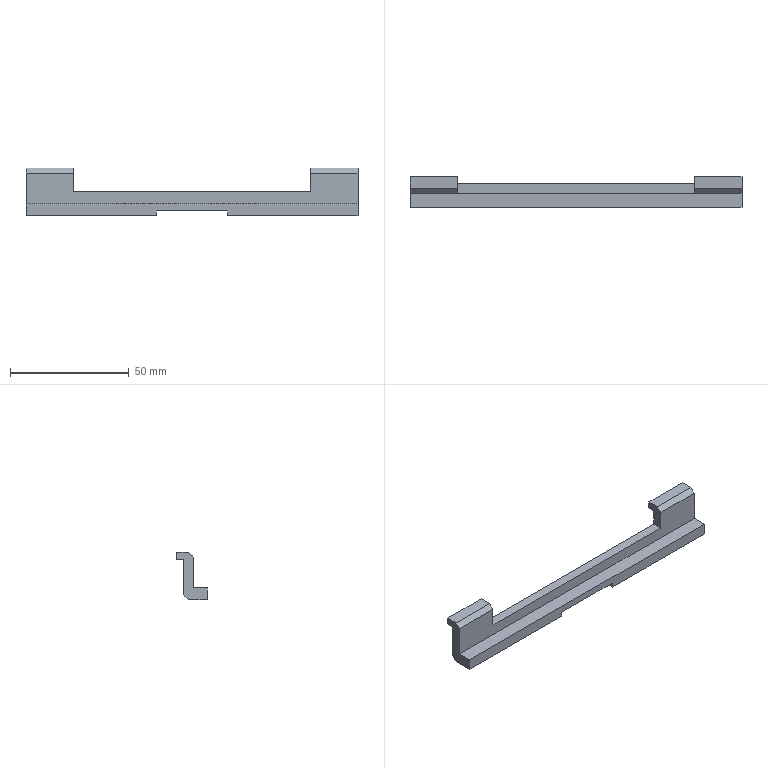Component | SolidWorks | Gripper-2024-3-4-07-1 | 1 solid | 24 faces | box 140 x 13 x 20 mm | volume 10860 mm3 | plane 24 | material S45C
build123d program:
from build123d import *

# Parameters (mm, degrees)
BOSS_EXTRUDE1_DEPTH = 140
SKETCH2_W           = 100
SKETCH2_H           = 10
CUT_EXTRUDE1_DEPTH  = 250
SKETCH3_W           = 10
SKETCH3_H           = 30
CUT_EXTRUDE2_DEPTH  = 2
SKETCH4_W           = 6
SKETCH4_H           = 15
CUT_EXTRUDE3_DEPTH  = 143.018
CHAMFER1_SIZE       = 2


with BuildPart() as part:
    # Sketch1 → Boss-Extrude1 (new body)
    with BuildSketch(Plane.XY):
        Polygon((0, 0), (-13, 0), (-13, 3), (-10, 3), (-10, 20), (0, 20), align=None)
    extrude(amount=BOSS_EXTRUDE1_DEPTH)

    # Sketch2 → Cut-Extrude1 (cut)
    with BuildSketch(Plane(origin=(0, 0, 0), x_dir=(0, 0, -1), z_dir=(1, 0, 0))):
        with Locations((-70, 5)):
            Rectangle(SKETCH2_W, SKETCH2_H)
    extrude(amount=-CUT_EXTRUDE1_DEPTH, mode=Mode.SUBTRACT)

    # Sketch3 → Cut-Extrude2 (cut)
    with BuildSketch(Plane(origin=(0, 20, 0), x_dir=(1, 0, 0), z_dir=(0, 1, 0))):
        with Locations((-5, -70)):
            Rectangle(SKETCH3_W, SKETCH3_H)
    extrude(amount=-CUT_EXTRUDE2_DEPTH, mode=Mode.SUBTRACT)

    # Sketch4 → Cut-Extrude3 (cut, through all)
    with BuildSketch(Plane.XY.offset(140)):
        with Locations((-3, 7.5)):
            Rectangle(SKETCH4_W, SKETCH4_H)
    extrude(amount=-CUT_EXTRUDE3_DEPTH, mode=Mode.SUBTRACT)

    # Chamfer1
    chamfer1_edges = [part.edges().sort_by_distance(p)[0] for p in [
        (-10, 20, 27.5),
        (-10, 20, 112.5),
        (-6, 0, 10),
        (-6, 0, 130),
    ]]
    chamfer(chamfer1_edges, length=CHAMFER1_SIZE)


solid = part.part

# Placed as in the assembly
solid = solid.moved(Location((-170.094, -141.769, 348), (-90, 90, 0)))
STEP:
#1=COLOUR_RGB('',0.7922,0.8196,0.9333);
#2=FILL_AREA_STYLE_COLOUR('',#1);
#3=FILL_AREA_STYLE('',(#2));
#4=SURFACE_STYLE_FILL_AREA(#3);
#5=SURFACE_SIDE_STYLE('',(#4));
#6=SURFACE_STYLE_USAGE(.BOTH.,#5);
#7=PRESENTATION_STYLE_ASSIGNMENT((#6));
#8=CARTESIAN_POINT('',(-6.697,-5.581,12.913));
#9=VERTEX_POINT('',#8);
#10=CARTESIAN_POINT('',(-6.697,-5.267,12.913));
#11=VERTEX_POINT('',#10);
#12=CARTESIAN_POINT('',(-6.697,-5.581,12.913));
#13=DIRECTION('',(-0.,1.,-0.));
#14=VECTOR('',#13,39.37);
#15=LINE('',#12,#14);
#16=EDGE_CURVE('',#9,#11,#15,.T.);
#17=ORIENTED_EDGE('',*,*,#16,.T.);
#18=CARTESIAN_POINT('',(-4.531,-5.267,12.913));
#19=VERTEX_POINT('',#18);
#20=CARTESIAN_POINT('',(-1.185,-5.267,12.913));
#21=DIRECTION('',(1.,-0.,0.));
#22=VECTOR('',#21,39.37);
#23=LINE('',#20,#22);
#24=EDGE_CURVE('',#11,#19,#23,.T.);
#25=ORIENTED_EDGE('',*,*,#24,.T.);
#26=CARTESIAN_POINT('',(-4.531,-5.581,12.913));
#27=VERTEX_POINT('',#26);
#28=CARTESIAN_POINT('',(-4.531,-5.581,12.913));
#29=DIRECTION('',(-0.,1.,-0.));
#30=VECTOR('',#29,39.37);
#31=LINE('',#28,#30);
#32=EDGE_CURVE('',#27,#19,#31,.T.);
#33=ORIENTED_EDGE('',*,*,#32,.F.);
#34=CARTESIAN_POINT('',(-1.185,-5.581,12.913));
#35=DIRECTION('',(-1.,0.,-0.));
#36=VECTOR('',#35,39.37);
#37=LINE('',#34,#36);
#38=EDGE_CURVE('',#27,#9,#37,.T.);
#39=ORIENTED_EDGE('',*,*,#38,.T.);
#40=EDGE_LOOP('',(#17,#25,#33,#39));
#41=FACE_OUTER_BOUND('',#40,.T.);
#42=CARTESIAN_POINT('',(-1.185,-5.581,12.913));
#43=DIRECTION('',(-0.,0.,1.));
#44=DIRECTION('',(0.,-1.,0.));
#45=AXIS2_PLACEMENT_3D('',#42,#43,#44);
#46=PLANE('',#45);
#47=ADVANCED_FACE('',(#41),#46,.F.);
#48=CARTESIAN_POINT('',(-1.185,-5.188,13.583));
#49=VERTEX_POINT('',#48);
#50=CARTESIAN_POINT('',(-1.972,-5.188,13.583));
#51=VERTEX_POINT('',#50);
#52=CARTESIAN_POINT('',(-1.185,-5.188,13.583));
#53=DIRECTION('',(-1.,0.,-0.));
#54=VECTOR('',#53,39.37);
#55=LINE('',#52,#54);
#56=EDGE_CURVE('',#49,#51,#55,.T.);
#57=ORIENTED_EDGE('',*,*,#56,.T.);
#58=CARTESIAN_POINT('',(-1.972,-5.07,13.583));
#59=VERTEX_POINT('',#58);
#60=CARTESIAN_POINT('',(-1.972,-5.07,13.583));
#61=DIRECTION('',(-0.,1.,-0.));
#62=VECTOR('',#61,39.37);
#63=LINE('',#60,#62);
#64=EDGE_CURVE('',#51,#59,#63,.T.);
#65=ORIENTED_EDGE('',*,*,#64,.T.);
#66=CARTESIAN_POINT('',(-1.185,-5.07,13.583));
#67=VERTEX_POINT('',#66);
#68=CARTESIAN_POINT('',(-1.185,-5.07,13.583));
#69=DIRECTION('',(-1.,0.,-0.));
#70=VECTOR('',#69,39.37);
#71=LINE('',#68,#70);
#72=EDGE_CURVE('',#67,#59,#71,.T.);
#73=ORIENTED_EDGE('',*,*,#72,.F.);
#74=CARTESIAN_POINT('',(-1.185,-5.07,13.583));
#75=DIRECTION('',(-0.,1.,-0.));
#76=VECTOR('',#75,39.37);
#77=LINE('',#74,#76);
#78=EDGE_CURVE('',#49,#67,#77,.T.);
#79=ORIENTED_EDGE('',*,*,#78,.F.);
#80=EDGE_LOOP('',(#57,#65,#73,#79));
#81=FACE_OUTER_BOUND('',#80,.T.);
#82=CARTESIAN_POINT('',(-1.185,-5.07,13.583));
#83=DIRECTION('',(-0.,0.,1.));
#84=DIRECTION('',(-1.,0.,-0.));
#85=AXIS2_PLACEMENT_3D('',#82,#83,#84);
#86=PLANE('',#85);
#87=ADVANCED_FACE('',(#81),#86,.F.);
#88=ORIENTED_EDGE('',*,*,#72,.T.);
#89=CARTESIAN_POINT('',(-1.972,-5.07,13.701));
#90=VERTEX_POINT('',#89);
#91=CARTESIAN_POINT('',(-1.972,-5.07,13.701));
#92=DIRECTION('',(-0.,0.,1.));
#93=VECTOR('',#92,39.37);
#94=LINE('',#91,#93);
#95=EDGE_CURVE('',#59,#90,#94,.T.);
#96=ORIENTED_EDGE('',*,*,#95,.T.);
#97=CARTESIAN_POINT('',(-1.185,-5.07,13.701));
#98=VERTEX_POINT('',#97);
#99=CARTESIAN_POINT('',(-1.185,-5.07,13.701));
#100=DIRECTION('',(-1.,0.,-0.));
#101=VECTOR('',#100,39.37);
#102=LINE('',#99,#101);
#103=EDGE_CURVE('',#98,#90,#102,.T.);
#104=ORIENTED_EDGE('',*,*,#103,.F.);
#105=CARTESIAN_POINT('',(-1.185,-5.07,13.701));
#106=DIRECTION('',(-0.,0.,1.));
#107=VECTOR('',#106,39.37);
#108=LINE('',#105,#107);
#109=EDGE_CURVE('',#67,#98,#108,.T.);
#110=ORIENTED_EDGE('',*,*,#109,.F.);
#111=EDGE_LOOP('',(#88,#96,#104,#110));
#112=FACE_OUTER_BOUND('',#111,.T.);
#113=CARTESIAN_POINT('',(-1.185,-5.07,13.701));
#114=DIRECTION('',(-0.,-1.,0.));
#115=DIRECTION('',(-1.,0.,-0.));
#116=AXIS2_PLACEMENT_3D('',#113,#114,#115);
#117=PLANE('',#116);
#118=ADVANCED_FACE('',(#112),#117,.F.);
#119=CARTESIAN_POINT('',(-1.972,-5.267,13.701));
#120=VERTEX_POINT('',#119);
#121=CARTESIAN_POINT('',(-1.972,-5.581,13.701));
#122=DIRECTION('',(0.,-1.,-0.));
#123=VECTOR('',#122,39.37);
#124=LINE('',#121,#123);
#125=EDGE_CURVE('',#90,#120,#124,.T.);
#126=ORIENTED_EDGE('',*,*,#125,.T.);
#127=CARTESIAN_POINT('',(-1.185,-5.267,13.701));
#128=VERTEX_POINT('',#127);
#129=CARTESIAN_POINT('',(-1.185,-5.267,13.701));
#130=DIRECTION('',(1.,-0.,0.));
#131=VECTOR('',#130,39.37);
#132=LINE('',#129,#131);
#133=EDGE_CURVE('',#120,#128,#132,.T.);
#134=ORIENTED_EDGE('',*,*,#133,.T.);
#135=CARTESIAN_POINT('',(-1.185,-5.581,13.701));
#136=DIRECTION('',(0.,-1.,-0.));
#137=VECTOR('',#136,39.37);
#138=LINE('',#135,#137);
#139=EDGE_CURVE('',#98,#128,#138,.T.);
#140=ORIENTED_EDGE('',*,*,#139,.F.);
#141=ORIENTED_EDGE('',*,*,#103,.T.);
#142=EDGE_LOOP('',(#126,#134,#140,#141));
#143=FACE_OUTER_BOUND('',#142,.T.);
#144=CARTESIAN_POINT('',(-1.185,-5.581,13.701));
#145=DIRECTION('',(0.,0.,-1.));
#146=DIRECTION('',(-0.,1.,0.));
#147=AXIS2_PLACEMENT_3D('',#144,#145,#146);
#148=PLANE('',#147);
#149=ADVANCED_FACE('',(#143),#148,.F.);
#150=CARTESIAN_POINT('',(-1.185,-5.581,13.11));
#151=VERTEX_POINT('',#150);
#152=CARTESIAN_POINT('',(-1.185,-5.581,12.913));
#153=VERTEX_POINT('',#152);
#154=CARTESIAN_POINT('',(-1.185,-5.581,13.701));
#155=DIRECTION('',(0.,-0.,-1.));
#156=VECTOR('',#155,39.37);
#157=LINE('',#154,#156);
#158=EDGE_CURVE('',#151,#153,#157,.T.);
#159=ORIENTED_EDGE('',*,*,#158,.F.);
#160=CARTESIAN_POINT('',(-6.697,-5.581,13.11));
#161=VERTEX_POINT('',#160);
#162=CARTESIAN_POINT('',(-6.697,-5.581,13.11));
#163=DIRECTION('',(1.,-0.,0.));
#164=VECTOR('',#163,39.37);
#165=LINE('',#162,#164);
#166=EDGE_CURVE('',#161,#151,#165,.T.);
#167=ORIENTED_EDGE('',*,*,#166,.F.);
#168=CARTESIAN_POINT('',(-6.697,-5.581,13.701));
#169=DIRECTION('',(0.,-0.,-1.));
#170=VECTOR('',#169,39.37);
#171=LINE('',#168,#170);
#172=EDGE_CURVE('',#161,#9,#171,.T.);
#173=ORIENTED_EDGE('',*,*,#172,.T.);
#174=ORIENTED_EDGE('',*,*,#38,.F.);
#175=CARTESIAN_POINT('',(-4.531,-5.581,12.992));
#176=VERTEX_POINT('',#175);
#177=CARTESIAN_POINT('',(-4.531,-5.581,12.992));
#178=DIRECTION('',(0.,-0.,-1.));
#179=VECTOR('',#178,39.37);
#180=LINE('',#177,#179);
#181=EDGE_CURVE('',#176,#27,#180,.T.);
#182=ORIENTED_EDGE('',*,*,#181,.F.);
#183=CARTESIAN_POINT('',(-3.35,-5.581,12.992));
#184=VERTEX_POINT('',#183);
#185=CARTESIAN_POINT('',(-3.35,-5.581,12.992));
#186=DIRECTION('',(-1.,0.,-0.));
#187=VECTOR('',#186,39.37);
#188=LINE('',#185,#187);
#189=EDGE_CURVE('',#184,#176,#188,.T.);
#190=ORIENTED_EDGE('',*,*,#189,.F.);
#191=CARTESIAN_POINT('',(-3.35,-5.581,12.913));
#192=VERTEX_POINT('',#191);
#193=CARTESIAN_POINT('',(-3.35,-5.581,12.992));
#194=DIRECTION('',(0.,-0.,-1.));
#195=VECTOR('',#194,39.37);
#196=LINE('',#193,#195);
#197=EDGE_CURVE('',#184,#192,#196,.T.);
#198=ORIENTED_EDGE('',*,*,#197,.T.);
#199=CARTESIAN_POINT('',(-1.185,-5.581,12.913));
#200=DIRECTION('',(-1.,0.,-0.));
#201=VECTOR('',#200,39.37);
#202=LINE('',#199,#201);
#203=EDGE_CURVE('',#153,#192,#202,.T.);
#204=ORIENTED_EDGE('',*,*,#203,.F.);
#205=EDGE_LOOP('',(#159,#167,#173,#174,#182,#190,#198,#204));
#206=FACE_OUTER_BOUND('',#205,.T.);
#207=CARTESIAN_POINT('',(-1.185,-5.581,13.701));
#208=DIRECTION('',(0.,1.,-0.));
#209=DIRECTION('',(1.,-0.,0.));
#210=AXIS2_PLACEMENT_3D('',#207,#208,#209);
#211=PLANE('',#210);
#212=ADVANCED_FACE('',(#206),#211,.F.);
#213=CARTESIAN_POINT('',(-3.35,-5.267,12.913));
#214=VERTEX_POINT('',#213);
#215=CARTESIAN_POINT('',(-3.35,-5.581,12.913));
#216=DIRECTION('',(0.,-1.,0.));
#217=VECTOR('',#216,39.37);
#218=LINE('',#215,#217);
#219=EDGE_CURVE('',#214,#192,#218,.T.);
#220=ORIENTED_EDGE('',*,*,#219,.F.);
#221=CARTESIAN_POINT('',(-1.185,-5.267,12.913));
#222=VERTEX_POINT('',#221);
#223=CARTESIAN_POINT('',(-1.185,-5.267,12.913));
#224=DIRECTION('',(1.,-0.,0.));
#225=VECTOR('',#224,39.37);
#226=LINE('',#223,#225);
#227=EDGE_CURVE('',#214,#222,#226,.T.);
#228=ORIENTED_EDGE('',*,*,#227,.T.);
#229=CARTESIAN_POINT('',(-1.185,-5.581,12.913));
#230=DIRECTION('',(-0.,1.,-0.));
#231=VECTOR('',#230,39.37);
#232=LINE('',#229,#231);
#233=EDGE_CURVE('',#153,#222,#232,.T.);
#234=ORIENTED_EDGE('',*,*,#233,.F.);
#235=ORIENTED_EDGE('',*,*,#203,.T.);
#236=EDGE_LOOP('',(#220,#228,#234,#235));
#237=FACE_OUTER_BOUND('',#236,.T.);
#238=CARTESIAN_POINT('',(-1.185,-5.581,12.913));
#239=DIRECTION('',(-0.,0.,1.));
#240=DIRECTION('',(0.,-1.,0.));
#241=AXIS2_PLACEMENT_3D('',#238,#239,#240);
#242=PLANE('',#241);
#243=ADVANCED_FACE('',(#237),#242,.F.);
#244=CARTESIAN_POINT('',(-4.531,-5.188,12.992));
#245=VERTEX_POINT('',#244);
#246=CARTESIAN_POINT('',(-3.35,-5.188,12.992));
#247=VERTEX_POINT('',#246);
#248=CARTESIAN_POINT('',(-3.35,-5.188,12.992));
#249=DIRECTION('',(1.,-0.,0.));
#250=VECTOR('',#249,39.37);
#251=LINE('',#248,#250);
#252=EDGE_CURVE('',#245,#247,#251,.T.);
#253=ORIENTED_EDGE('',*,*,#252,.F.);
#254=CARTESIAN_POINT('',(-6.697,-5.188,12.992));
#255=VERTEX_POINT('',#254);
#256=CARTESIAN_POINT('',(-1.185,-5.188,12.992));
#257=DIRECTION('',(-1.,0.,-0.));
#258=VECTOR('',#257,39.37);
#259=LINE('',#256,#258);
#260=EDGE_CURVE('',#245,#255,#259,.T.);
#261=ORIENTED_EDGE('',*,*,#260,.T.);
#262=CARTESIAN_POINT('',(-6.697,-5.188,13.583));
#263=VERTEX_POINT('',#262);
#264=CARTESIAN_POINT('',(-6.697,-5.188,12.913));
#265=DIRECTION('',(-0.,-0.,1.));
#266=VECTOR('',#265,39.37);
#267=LINE('',#264,#266);
#268=EDGE_CURVE('',#255,#263,#267,.T.);
#269=ORIENTED_EDGE('',*,*,#268,.T.);
#270=CARTESIAN_POINT('',(-5.909,-5.188,13.583));
#271=VERTEX_POINT('',#270);
#272=CARTESIAN_POINT('',(-1.185,-5.188,13.583));
#273=DIRECTION('',(-1.,0.,-0.));
#274=VECTOR('',#273,39.37);
#275=LINE('',#272,#274);
#276=EDGE_CURVE('',#271,#263,#275,.T.);
#277=ORIENTED_EDGE('',*,*,#276,.F.);
#278=CARTESIAN_POINT('',(-5.909,-5.188,13.307));
#279=VERTEX_POINT('',#278);
#280=CARTESIAN_POINT('',(-5.909,-5.188,12.913));
#281=DIRECTION('',(0.,0.,-1.));
#282=VECTOR('',#281,39.37);
#283=LINE('',#280,#282);
#284=EDGE_CURVE('',#271,#279,#283,.T.);
#285=ORIENTED_EDGE('',*,*,#284,.T.);
#286=CARTESIAN_POINT('',(-1.972,-5.188,13.307));
#287=VERTEX_POINT('',#286);
#288=CARTESIAN_POINT('',(-1.185,-5.188,13.307));
#289=DIRECTION('',(1.,-0.,0.));
#290=VECTOR('',#289,39.37);
#291=LINE('',#288,#290);
#292=EDGE_CURVE('',#279,#287,#291,.T.);
#293=ORIENTED_EDGE('',*,*,#292,.T.);
#294=CARTESIAN_POINT('',(-1.972,-5.188,12.913));
#295=DIRECTION('',(-0.,-0.,1.));
#296=VECTOR('',#295,39.37);
#297=LINE('',#294,#296);
#298=EDGE_CURVE('',#287,#51,#297,.T.);
#299=ORIENTED_EDGE('',*,*,#298,.T.);
#300=ORIENTED_EDGE('',*,*,#56,.F.);
#301=CARTESIAN_POINT('',(-1.185,-5.188,12.992));
#302=VERTEX_POINT('',#301);
#303=CARTESIAN_POINT('',(-1.185,-5.188,12.913));
#304=DIRECTION('',(-0.,-0.,1.));
#305=VECTOR('',#304,39.37);
#306=LINE('',#303,#305);
#307=EDGE_CURVE('',#302,#49,#306,.T.);
#308=ORIENTED_EDGE('',*,*,#307,.F.);
#309=CARTESIAN_POINT('',(-1.185,-5.188,12.992));
#310=DIRECTION('',(-1.,0.,-0.));
#311=VECTOR('',#310,39.37);
#312=LINE('',#309,#311);
#313=EDGE_CURVE('',#302,#247,#312,.T.);
#314=ORIENTED_EDGE('',*,*,#313,.T.);
#315=EDGE_LOOP('',(#253,#261,#269,#277,#285,#293,#299,#300,#308,#314));
#316=FACE_OUTER_BOUND('',#315,.T.);
#317=CARTESIAN_POINT('',(-1.185,-5.188,12.913));
#318=DIRECTION('',(0.,-1.,-0.));
#319=DIRECTION('',(0.,0.,-1.));
#320=AXIS2_PLACEMENT_3D('',#317,#318,#319);
#321=PLANE('',#320);
#322=ADVANCED_FACE('',(#316),#321,.F.);
#323=CARTESIAN_POINT('',(-5.909,-5.07,13.583));
#324=VERTEX_POINT('',#323);
#325=CARTESIAN_POINT('',(-6.697,-5.07,13.583));
#326=VERTEX_POINT('',#325);
#327=CARTESIAN_POINT('',(-1.185,-5.07,13.583));
#328=DIRECTION('',(-1.,0.,-0.));
#329=VECTOR('',#328,39.37);
#330=LINE('',#327,#329);
#331=EDGE_CURVE('',#324,#326,#330,.T.);
#332=ORIENTED_EDGE('',*,*,#331,.F.);
#333=CARTESIAN_POINT('',(-5.909,-5.07,13.583));
#334=DIRECTION('',(0.,-1.,0.));
#335=VECTOR('',#334,39.37);
#336=LINE('',#333,#335);
#337=EDGE_CURVE('',#324,#271,#336,.T.);
#338=ORIENTED_EDGE('',*,*,#337,.T.);
#339=ORIENTED_EDGE('',*,*,#276,.T.);
#340=CARTESIAN_POINT('',(-6.697,-5.07,13.583));
#341=DIRECTION('',(-0.,1.,-0.));
#342=VECTOR('',#341,39.37);
#343=LINE('',#340,#342);
#344=EDGE_CURVE('',#263,#326,#343,.T.);
#345=ORIENTED_EDGE('',*,*,#344,.T.);
#346=EDGE_LOOP('',(#332,#338,#339,#345));
#347=FACE_OUTER_BOUND('',#346,.T.);
#348=CARTESIAN_POINT('',(-1.185,-5.07,13.583));
#349=DIRECTION('',(-0.,0.,1.));
#350=DIRECTION('',(-1.,0.,-0.));
#351=AXIS2_PLACEMENT_3D('',#348,#349,#350);
#352=PLANE('',#351);
#353=ADVANCED_FACE('',(#347),#352,.F.);
#354=CARTESIAN_POINT('',(-5.909,-5.07,13.701));
#355=VERTEX_POINT('',#354);
#356=CARTESIAN_POINT('',(-6.697,-5.07,13.701));
#357=VERTEX_POINT('',#356);
#358=CARTESIAN_POINT('',(-1.185,-5.07,13.701));
#359=DIRECTION('',(-1.,0.,-0.));
#360=VECTOR('',#359,39.37);
#361=LINE('',#358,#360);
#362=EDGE_CURVE('',#355,#357,#361,.T.);
#363=ORIENTED_EDGE('',*,*,#362,.F.);
#364=CARTESIAN_POINT('',(-5.909,-5.07,13.701));
#365=DIRECTION('',(0.,-0.,-1.));
#366=VECTOR('',#365,39.37);
#367=LINE('',#364,#366);
#368=EDGE_CURVE('',#355,#324,#367,.T.);
#369=ORIENTED_EDGE('',*,*,#368,.T.);
#370=ORIENTED_EDGE('',*,*,#331,.T.);
#371=CARTESIAN_POINT('',(-6.697,-5.07,13.701));
#372=DIRECTION('',(-0.,0.,1.));
#373=VECTOR('',#372,39.37);
#374=LINE('',#371,#373);
#375=EDGE_CURVE('',#326,#357,#374,.T.);
#376=ORIENTED_EDGE('',*,*,#375,.T.);
#377=EDGE_LOOP('',(#363,#369,#370,#376));
#378=FACE_OUTER_BOUND('',#377,.T.);
#379=CARTESIAN_POINT('',(-1.185,-5.07,13.701));
#380=DIRECTION('',(-0.,-1.,0.));
#381=DIRECTION('',(-1.,0.,-0.));
#382=AXIS2_PLACEMENT_3D('',#379,#380,#381);
#383=PLANE('',#382);
#384=ADVANCED_FACE('',(#378),#383,.F.);
#385=CARTESIAN_POINT('',(-6.697,-5.267,13.701));
#386=VERTEX_POINT('',#385);
#387=CARTESIAN_POINT('',(-6.697,-5.581,13.701));
#388=DIRECTION('',(0.,-1.,-0.));
#389=VECTOR('',#388,39.37);
#390=LINE('',#387,#389);
#391=EDGE_CURVE('',#357,#386,#390,.T.);
#392=ORIENTED_EDGE('',*,*,#391,.T.);
#393=CARTESIAN_POINT('',(-5.909,-5.267,13.701));
#394=VERTEX_POINT('',#393);
#395=CARTESIAN_POINT('',(-1.185,-5.267,13.701));
#396=DIRECTION('',(1.,-0.,0.));
#397=VECTOR('',#396,39.37);
#398=LINE('',#395,#397);
#399=EDGE_CURVE('',#386,#394,#398,.T.);
#400=ORIENTED_EDGE('',*,*,#399,.T.);
#401=CARTESIAN_POINT('',(-5.909,-5.581,13.701));
#402=DIRECTION('',(-0.,1.,0.));
#403=VECTOR('',#402,39.37);
#404=LINE('',#401,#403);
#405=EDGE_CURVE('',#394,#355,#404,.T.);
#406=ORIENTED_EDGE('',*,*,#405,.T.);
#407=ORIENTED_EDGE('',*,*,#362,.T.);
#408=EDGE_LOOP('',(#392,#400,#406,#407));
#409=FACE_OUTER_BOUND('',#408,.T.);
#410=CARTESIAN_POINT('',(-1.185,-5.581,13.701));
#411=DIRECTION('',(0.,0.,-1.));
#412=DIRECTION('',(-0.,1.,0.));
#413=AXIS2_PLACEMENT_3D('',#410,#411,#412);
#414=PLANE('',#413);
#415=ADVANCED_FACE('',(#409),#414,.F.);
#416=ORIENTED_EDGE('',*,*,#233,.T.);
#417=CARTESIAN_POINT('',(-1.185,-5.03,13.15));
#418=DIRECTION('',(-0.,0.7071,0.7071));
#419=VECTOR('',#418,39.37);
#420=LINE('',#417,#419);
#421=EDGE_CURVE('',#222,#302,#420,.T.);
#422=ORIENTED_EDGE('',*,*,#421,.T.);
#423=ORIENTED_EDGE('',*,*,#307,.T.);
#424=ORIENTED_EDGE('',*,*,#78,.T.);
#425=ORIENTED_EDGE('',*,*,#109,.T.);
#426=ORIENTED_EDGE('',*,*,#139,.T.);
#427=CARTESIAN_POINT('',(-1.185,-5.345,13.622));
#428=VERTEX_POINT('',#427);
#429=CARTESIAN_POINT('',(-1.185,-5.424,13.543));
#430=DIRECTION('',(0.,-0.7071,-0.7071));
#431=VECTOR('',#430,39.37);
#432=LINE('',#429,#431);
#433=EDGE_CURVE('',#128,#428,#432,.T.);
#434=ORIENTED_EDGE('',*,*,#433,.T.);
#435=CARTESIAN_POINT('',(-1.185,-5.345,13.11));
#436=VERTEX_POINT('',#435);
#437=CARTESIAN_POINT('',(-1.185,-5.345,13.701));
#438=DIRECTION('',(-0.,0.,1.));
#439=VECTOR('',#438,39.37);
#440=LINE('',#437,#439);
#441=EDGE_CURVE('',#436,#428,#440,.T.);
#442=ORIENTED_EDGE('',*,*,#441,.F.);
#443=CARTESIAN_POINT('',(-1.185,-5.581,13.11));
#444=DIRECTION('',(-0.,1.,-0.));
#445=VECTOR('',#444,39.37);
#446=LINE('',#443,#445);
#447=EDGE_CURVE('',#151,#436,#446,.T.);
#448=ORIENTED_EDGE('',*,*,#447,.F.);
#449=ORIENTED_EDGE('',*,*,#158,.T.);
#450=EDGE_LOOP('',(#416,#422,#423,#424,#425,#426,#434,#442,#448,#449));
#451=FACE_OUTER_BOUND('',#450,.T.);
#452=CARTESIAN_POINT('',(-1.185,-5.581,13.701));
#453=DIRECTION('',(1.,0.,0.));
#454=DIRECTION('',(0.,-1.,0.));
#455=AXIS2_PLACEMENT_3D('',#452,#453,#454);
#456=PLANE('',#455);
#457=ADVANCED_FACE('',(#451),#456,.T.);
#458=ORIENTED_EDGE('',*,*,#268,.F.);
#459=CARTESIAN_POINT('',(-6.697,-5.188,12.992));
#460=DIRECTION('',(0.,-0.7071,-0.7071));
#461=VECTOR('',#460,39.37);
#462=LINE('',#459,#461);
#463=EDGE_CURVE('',#255,#11,#462,.T.);
#464=ORIENTED_EDGE('',*,*,#463,.T.);
#465=ORIENTED_EDGE('',*,*,#16,.F.);
#466=ORIENTED_EDGE('',*,*,#172,.F.);
#467=CARTESIAN_POINT('',(-6.697,-5.345,13.11));
#468=VERTEX_POINT('',#467);
#469=CARTESIAN_POINT('',(-6.697,-5.581,13.11));
#470=DIRECTION('',(-0.,1.,-0.));
#471=VECTOR('',#470,39.37);
#472=LINE('',#469,#471);
#473=EDGE_CURVE('',#161,#468,#472,.T.);
#474=ORIENTED_EDGE('',*,*,#473,.T.);
#475=CARTESIAN_POINT('',(-6.697,-5.345,13.622));
#476=VERTEX_POINT('',#475);
#477=CARTESIAN_POINT('',(-6.697,-5.345,13.701));
#478=DIRECTION('',(-0.,0.,1.));
#479=VECTOR('',#478,39.37);
#480=LINE('',#477,#479);
#481=EDGE_CURVE('',#468,#476,#480,.T.);
#482=ORIENTED_EDGE('',*,*,#481,.T.);
#483=CARTESIAN_POINT('',(-6.697,-5.267,13.701));
#484=DIRECTION('',(-0.,0.7071,0.7071));
#485=VECTOR('',#484,39.37);
#486=LINE('',#483,#485);
#487=EDGE_CURVE('',#476,#386,#486,.T.);
#488=ORIENTED_EDGE('',*,*,#487,.T.);
#489=ORIENTED_EDGE('',*,*,#391,.F.);
#490=ORIENTED_EDGE('',*,*,#375,.F.);
#491=ORIENTED_EDGE('',*,*,#344,.F.);
#492=EDGE_LOOP('',(#458,#464,#465,#466,#474,#482,#488,#489,#490,#491));
#493=FACE_OUTER_BOUND('',#492,.T.);
#494=CARTESIAN_POINT('',(-6.697,-5.581,13.701));
#495=DIRECTION('',(1.,0.,0.));
#496=DIRECTION('',(0.,-1.,0.));
#497=AXIS2_PLACEMENT_3D('',#494,#495,#496);
#498=PLANE('',#497);
#499=ADVANCED_FACE('',(#493),#498,.F.);
#500=CARTESIAN_POINT('',(-5.909,-5.345,13.307));
#501=VERTEX_POINT('',#500);
#502=CARTESIAN_POINT('',(-5.909,4.261,13.307));
#503=DIRECTION('',(0.,-1.,0.));
#504=VECTOR('',#503,39.37);
#505=LINE('',#502,#504);
#506=EDGE_CURVE('',#279,#501,#505,.T.);
#507=ORIENTED_EDGE('',*,*,#506,.T.);
#508=CARTESIAN_POINT('',(-1.972,-5.345,13.307));
#509=VERTEX_POINT('',#508);
#510=CARTESIAN_POINT('',(-1.972,-5.345,13.307));
#511=DIRECTION('',(1.,-0.,0.));
#512=VECTOR('',#511,39.37);
#513=LINE('',#510,#512);
#514=EDGE_CURVE('',#501,#509,#513,.T.);
#515=ORIENTED_EDGE('',*,*,#514,.T.);
#516=CARTESIAN_POINT('',(-1.972,4.261,13.307));
#517=DIRECTION('',(0.,-1.,0.));
#518=VECTOR('',#517,39.37);
#519=LINE('',#516,#518);
#520=EDGE_CURVE('',#287,#509,#519,.T.);
#521=ORIENTED_EDGE('',*,*,#520,.F.);
#522=ORIENTED_EDGE('',*,*,#292,.F.);
#523=EDGE_LOOP('',(#507,#515,#521,#522));
#524=FACE_OUTER_BOUND('',#523,.T.);
#525=CARTESIAN_POINT('',(-1.972,4.261,13.307));
#526=DIRECTION('',(0.,-0.,-1.));
#527=DIRECTION('',(1.,-0.,0.));
#528=AXIS2_PLACEMENT_3D('',#525,#526,#527);
#529=PLANE('',#528);
#530=ADVANCED_FACE('',(#524),#529,.F.);
#531=CARTESIAN_POINT('',(-1.972,-5.345,13.622));
#532=VERTEX_POINT('',#531);
#533=CARTESIAN_POINT('',(-1.972,-5.345,13.701));
#534=DIRECTION('',(-0.,0.,1.));
#535=VECTOR('',#534,39.37);
#536=LINE('',#533,#535);
#537=EDGE_CURVE('',#509,#532,#536,.T.);
#538=ORIENTED_EDGE('',*,*,#537,.T.);
#539=CARTESIAN_POINT('',(-1.972,-5.267,13.701));
#540=DIRECTION('',(-0.,0.7071,0.7071));
#541=VECTOR('',#540,39.37);
#542=LINE('',#539,#541);
#543=EDGE_CURVE('',#532,#120,#542,.T.);
#544=ORIENTED_EDGE('',*,*,#543,.T.);
#545=ORIENTED_EDGE('',*,*,#125,.F.);
#546=ORIENTED_EDGE('',*,*,#95,.F.);
#547=ORIENTED_EDGE('',*,*,#64,.F.);
#548=ORIENTED_EDGE('',*,*,#298,.F.);
#549=ORIENTED_EDGE('',*,*,#520,.T.);
#550=EDGE_LOOP('',(#538,#544,#545,#546,#547,#548,#549));
#551=FACE_OUTER_BOUND('',#550,.T.);
#552=CARTESIAN_POINT('',(-1.972,4.261,13.701));
#553=DIRECTION('',(1.,0.,0.));
#554=DIRECTION('',(0.,-1.,0.));
#555=AXIS2_PLACEMENT_3D('',#552,#553,#554);
#556=PLANE('',#555);
#557=ADVANCED_FACE('',(#551),#556,.F.);
#558=ORIENTED_EDGE('',*,*,#405,.F.);
#559=CARTESIAN_POINT('',(-5.909,-5.345,13.622));
#560=VERTEX_POINT('',#559);
#561=CARTESIAN_POINT('',(-5.909,-5.267,13.701));
#562=DIRECTION('',(0.,-0.7071,-0.7071));
#563=VECTOR('',#562,39.37);
#564=LINE('',#561,#563);
#565=EDGE_CURVE('',#394,#560,#564,.T.);
#566=ORIENTED_EDGE('',*,*,#565,.T.);
#567=CARTESIAN_POINT('',(-5.909,-5.345,13.701));
#568=DIRECTION('',(0.,-0.,-1.));
#569=VECTOR('',#568,39.37);
#570=LINE('',#567,#569);
#571=EDGE_CURVE('',#560,#501,#570,.T.);
#572=ORIENTED_EDGE('',*,*,#571,.T.);
#573=ORIENTED_EDGE('',*,*,#506,.F.);
#574=ORIENTED_EDGE('',*,*,#284,.F.);
#575=ORIENTED_EDGE('',*,*,#337,.F.);
#576=ORIENTED_EDGE('',*,*,#368,.F.);
#577=EDGE_LOOP('',(#558,#566,#572,#573,#574,#575,#576));
#578=FACE_OUTER_BOUND('',#577,.T.);
#579=CARTESIAN_POINT('',(-5.909,4.261,13.701));
#580=DIRECTION('',(-1.,-0.,-0.));
#581=DIRECTION('',(-0.,1.,-0.));
#582=AXIS2_PLACEMENT_3D('',#579,#580,#581);
#583=PLANE('',#582);
#584=ADVANCED_FACE('',(#578),#583,.F.);
#585=ORIENTED_EDGE('',*,*,#32,.T.);
#586=CARTESIAN_POINT('',(-4.531,-5.188,12.992));
#587=DIRECTION('',(-0.,0.7071,0.7071));
#588=VECTOR('',#587,39.37);
#589=LINE('',#586,#588);
#590=EDGE_CURVE('',#19,#245,#589,.T.);
#591=ORIENTED_EDGE('',*,*,#590,.T.);
#592=CARTESIAN_POINT('',(-4.531,-5.581,12.992));
#593=DIRECTION('',(-0.,1.,-0.));
#594=VECTOR('',#593,39.37);
#595=LINE('',#592,#594);
#596=EDGE_CURVE('',#176,#245,#595,.T.);
#597=ORIENTED_EDGE('',*,*,#596,.F.);
#598=ORIENTED_EDGE('',*,*,#181,.T.);
#599=EDGE_LOOP('',(#585,#591,#597,#598));
#600=FACE_OUTER_BOUND('',#599,.T.);
#601=CARTESIAN_POINT('',(-4.531,-5.581,12.992));
#602=DIRECTION('',(-1.,-0.,-0.));
#603=DIRECTION('',(-0.,1.,-0.));
#604=AXIS2_PLACEMENT_3D('',#601,#602,#603);
#605=PLANE('',#604);
#606=ADVANCED_FACE('',(#600),#605,.F.);
#607=CARTESIAN_POINT('',(-3.35,-5.581,12.992));
#608=DIRECTION('',(0.,-1.,0.));
#609=VECTOR('',#608,39.37);
#610=LINE('',#607,#609);
#611=EDGE_CURVE('',#247,#184,#610,.T.);
#612=ORIENTED_EDGE('',*,*,#611,.F.);
#613=CARTESIAN_POINT('',(-3.35,-5.188,12.992));
#614=DIRECTION('',(0.,-0.7071,-0.7071));
#615=VECTOR('',#614,39.37);
#616=LINE('',#613,#615);
#617=EDGE_CURVE('',#247,#214,#616,.T.);
#618=ORIENTED_EDGE('',*,*,#617,.T.);
#619=ORIENTED_EDGE('',*,*,#219,.T.);
#620=ORIENTED_EDGE('',*,*,#197,.F.);
#621=EDGE_LOOP('',(#612,#618,#619,#620));
#622=FACE_OUTER_BOUND('',#621,.T.);
#623=CARTESIAN_POINT('',(-3.35,-5.581,12.992));
#624=DIRECTION('',(1.,0.,0.));
#625=DIRECTION('',(0.,-1.,0.));
#626=AXIS2_PLACEMENT_3D('',#623,#624,#625);
#627=PLANE('',#626);
#628=ADVANCED_FACE('',(#622),#627,.F.);
#629=ORIENTED_EDGE('',*,*,#252,.T.);
#630=ORIENTED_EDGE('',*,*,#611,.T.);
#631=ORIENTED_EDGE('',*,*,#189,.T.);
#632=ORIENTED_EDGE('',*,*,#596,.T.);
#633=EDGE_LOOP('',(#629,#630,#631,#632));
#634=FACE_OUTER_BOUND('',#633,.T.);
#635=CARTESIAN_POINT('',(-6.697,-5.581,12.992));
#636=DIRECTION('',(0.,-0.,-1.));
#637=DIRECTION('',(-0.,1.,-0.));
#638=AXIS2_PLACEMENT_3D('',#635,#636,#637);
#639=PLANE('',#638);
#640=ADVANCED_FACE('',(#634),#639,.T.);
#641=ORIENTED_EDGE('',*,*,#571,.F.);
#642=CARTESIAN_POINT('',(-6.697,-5.345,13.622));
#643=DIRECTION('',(-1.,0.,-0.));
#644=VECTOR('',#643,39.37);
#645=LINE('',#642,#644);
#646=EDGE_CURVE('',#560,#476,#645,.T.);
#647=ORIENTED_EDGE('',*,*,#646,.T.);
#648=ORIENTED_EDGE('',*,*,#481,.F.);
#649=CARTESIAN_POINT('',(-6.697,-5.345,13.11));
#650=DIRECTION('',(1.,-0.,0.));
#651=VECTOR('',#650,39.37);
#652=LINE('',#649,#651);
#653=EDGE_CURVE('',#468,#436,#652,.T.);
#654=ORIENTED_EDGE('',*,*,#653,.T.);
#655=ORIENTED_EDGE('',*,*,#441,.T.);
#656=CARTESIAN_POINT('',(-6.697,-5.345,13.622));
#657=DIRECTION('',(-1.,0.,-0.));
#658=VECTOR('',#657,39.37);
#659=LINE('',#656,#658);
#660=EDGE_CURVE('',#428,#532,#659,.T.);
#661=ORIENTED_EDGE('',*,*,#660,.T.);
#662=ORIENTED_EDGE('',*,*,#537,.F.);
#663=ORIENTED_EDGE('',*,*,#514,.F.);
#664=EDGE_LOOP('',(#641,#647,#648,#654,#655,#661,#662,#663));
#665=FACE_OUTER_BOUND('',#664,.T.);
#666=CARTESIAN_POINT('',(-6.697,-5.345,13.701));
#667=DIRECTION('',(0.,1.,-0.));
#668=DIRECTION('',(1.,-0.,0.));
#669=AXIS2_PLACEMENT_3D('',#666,#667,#668);
#670=PLANE('',#669);
#671=ADVANCED_FACE('',(#665),#670,.F.);
#672=ORIENTED_EDGE('',*,*,#447,.T.);
#673=ORIENTED_EDGE('',*,*,#653,.F.);
#674=ORIENTED_EDGE('',*,*,#473,.F.);
#675=ORIENTED_EDGE('',*,*,#166,.T.);
#676=EDGE_LOOP('',(#672,#673,#674,#675));
#677=FACE_OUTER_BOUND('',#676,.T.);
#678=CARTESIAN_POINT('',(-6.697,-5.581,13.11));
#679=DIRECTION('',(0.,-0.,-1.));
#680=DIRECTION('',(1.,-0.,0.));
#681=AXIS2_PLACEMENT_3D('',#678,#679,#680);
#682=PLANE('',#681);
#683=ADVANCED_FACE('',(#677),#682,.F.);
#684=ORIENTED_EDGE('',*,*,#590,.F.);
#685=ORIENTED_EDGE('',*,*,#24,.F.);
#686=ORIENTED_EDGE('',*,*,#463,.F.);
#687=ORIENTED_EDGE('',*,*,#260,.F.);
#688=EDGE_LOOP('',(#684,#685,#686,#687));
#689=FACE_OUTER_BOUND('',#688,.T.);
#690=CARTESIAN_POINT('',(-1.185,-5.188,12.992));
#691=DIRECTION('',(-0.,-0.7071,0.7071));
#692=DIRECTION('',(-1.,0.,-0.));
#693=AXIS2_PLACEMENT_3D('',#690,#691,#692);
#694=PLANE('',#693);
#695=ADVANCED_FACE('',(#689),#694,.F.);
#696=ORIENTED_EDGE('',*,*,#421,.F.);
#697=ORIENTED_EDGE('',*,*,#227,.F.);
#698=ORIENTED_EDGE('',*,*,#617,.F.);
#699=ORIENTED_EDGE('',*,*,#313,.F.);
#700=EDGE_LOOP('',(#696,#697,#698,#699));
#701=FACE_OUTER_BOUND('',#700,.T.);
#702=CARTESIAN_POINT('',(-1.185,-5.188,12.992));
#703=DIRECTION('',(-0.,-0.7071,0.7071));
#704=DIRECTION('',(-1.,0.,-0.));
#705=AXIS2_PLACEMENT_3D('',#702,#703,#704);
#706=PLANE('',#705);
#707=ADVANCED_FACE('',(#701),#706,.F.);
#708=ORIENTED_EDGE('',*,*,#487,.F.);
#709=ORIENTED_EDGE('',*,*,#646,.F.);
#710=ORIENTED_EDGE('',*,*,#565,.F.);
#711=ORIENTED_EDGE('',*,*,#399,.F.);
#712=EDGE_LOOP('',(#708,#709,#710,#711));
#713=FACE_OUTER_BOUND('',#712,.T.);
#714=CARTESIAN_POINT('',(-1.185,-5.267,13.701));
#715=DIRECTION('',(0.,0.7071,-0.7071));
#716=DIRECTION('',(1.,-0.,0.));
#717=AXIS2_PLACEMENT_3D('',#714,#715,#716);
#718=PLANE('',#717);
#719=ADVANCED_FACE('',(#713),#718,.F.);
#720=ORIENTED_EDGE('',*,*,#543,.F.);
#721=ORIENTED_EDGE('',*,*,#660,.F.);
#722=ORIENTED_EDGE('',*,*,#433,.F.);
#723=ORIENTED_EDGE('',*,*,#133,.F.);
#724=EDGE_LOOP('',(#720,#721,#722,#723));
#725=FACE_OUTER_BOUND('',#724,.T.);
#726=CARTESIAN_POINT('',(-1.185,-5.267,13.701));
#727=DIRECTION('',(0.,0.7071,-0.7071));
#728=DIRECTION('',(1.,-0.,0.));
#729=AXIS2_PLACEMENT_3D('',#726,#727,#728);
#730=PLANE('',#729);
#731=ADVANCED_FACE('',(#725),#730,.F.);
#732=CLOSED_SHELL('',(#47,#87,#118,#149,#212,#243,#322,#353,#384,#415,#457,#499,#530,#557,#584,#606,#628,#640,#671,#683,#695,#707,#719,#731));
#733=MANIFOLD_SOLID_BREP('',#732);
#734=STYLED_ITEM('',(#7),#733);
#735=(LENGTH_UNIT()NAMED_UNIT(*)SI_UNIT($,.METRE.));
#736=LENGTH_MEASURE_WITH_UNIT(LENGTH_MEASURE(0.0254),#735);
#737=DIMENSIONAL_EXPONENTS(1.,0.,0.,0.,0.,0.,0.);
#738=(CONVERSION_BASED_UNIT('',#736)LENGTH_UNIT()NAMED_UNIT(#737));
#739=UNCERTAINTY_MEASURE_WITH_UNIT(LENGTH_MEASURE(0.00001),#738,'','');
#740=(NAMED_UNIT(*)PLANE_ANGLE_UNIT()SI_UNIT($,.RADIAN.));
#741=(NAMED_UNIT(*)SI_UNIT($,.STERADIAN.)SOLID_ANGLE_UNIT());
#742=(GEOMETRIC_REPRESENTATION_CONTEXT(3)GLOBAL_UNCERTAINTY_ASSIGNED_CONTEXT((#739))GLOBAL_UNIT_ASSIGNED_CONTEXT((#738,#740,#741))REPRESENTATION_CONTEXT('',''));
#743=MECHANICAL_DESIGN_GEOMETRIC_PRESENTATION_REPRESENTATION('',(#734),#742);
#744=PRESENTATION_LAYER_ASSIGNMENT('','',(#734));
#745=CARTESIAN_POINT('',(0.,0.,0.));
#746=DIRECTION('',(0.,0.,1.));
#747=DIRECTION('',(1.,0.,0.));
#748=AXIS2_PLACEMENT_3D('',#745,#746,#747);
#749=(LENGTH_UNIT()NAMED_UNIT(*)SI_UNIT($,.METRE.));
#750=LENGTH_MEASURE_WITH_UNIT(LENGTH_MEASURE(0.0254),#749);
#751=DIMENSIONAL_EXPONENTS(1.,0.,0.,0.,0.,0.,0.);
#752=(CONVERSION_BASED_UNIT('',#750)LENGTH_UNIT()NAMED_UNIT(#751));
#753=UNCERTAINTY_MEASURE_WITH_UNIT(LENGTH_MEASURE(0.00001),#752,'','');
#754=(NAMED_UNIT(*)PLANE_ANGLE_UNIT()SI_UNIT($,.RADIAN.));
#755=(NAMED_UNIT(*)SI_UNIT($,.STERADIAN.)SOLID_ANGLE_UNIT());
#756=(GEOMETRIC_REPRESENTATION_CONTEXT(3)GLOBAL_UNCERTAINTY_ASSIGNED_CONTEXT((#753))GLOBAL_UNIT_ASSIGNED_CONTEXT((#752,#754,#755))REPRESENTATION_CONTEXT('',''));
#757=ADVANCED_BREP_SHAPE_REPRESENTATION('',(#733,#748),#756);